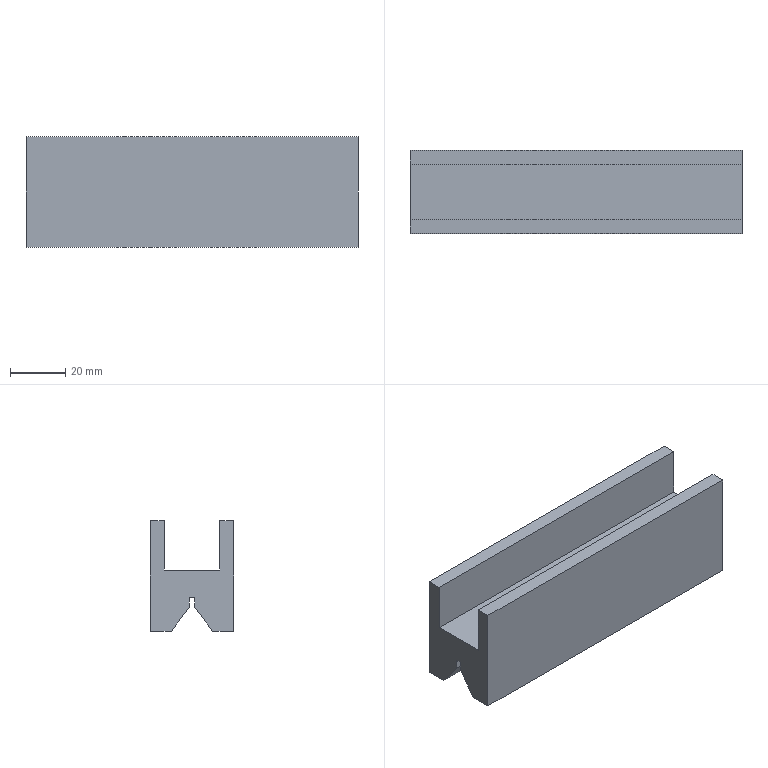CAM job | Mastercam | mm | 8 operations | part box 120 x 30 x 40
1. Contour (Ramp) | 2 - 12 平铣刀
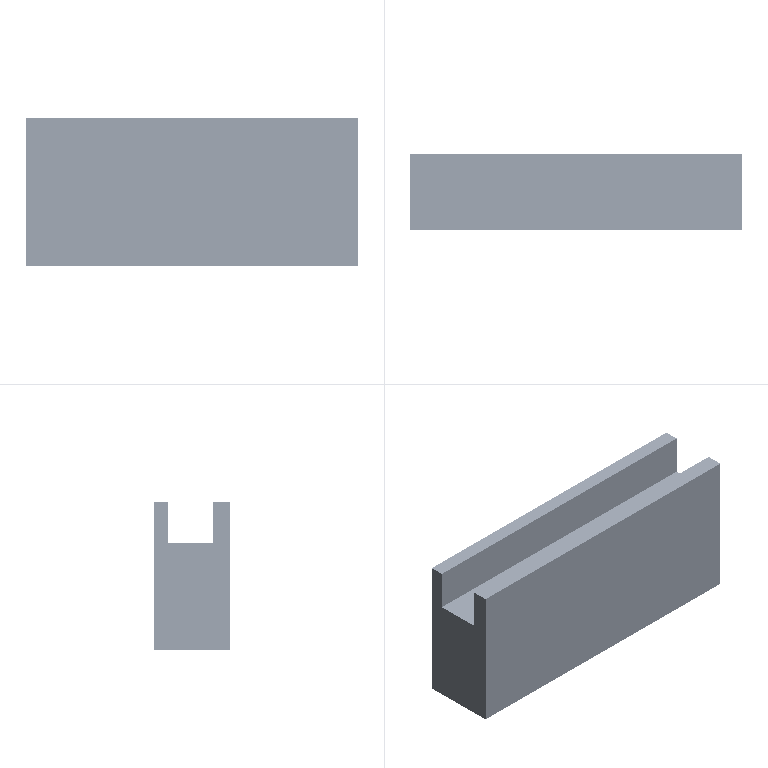2. Contour (2D) | 3 - 12 平铣刀
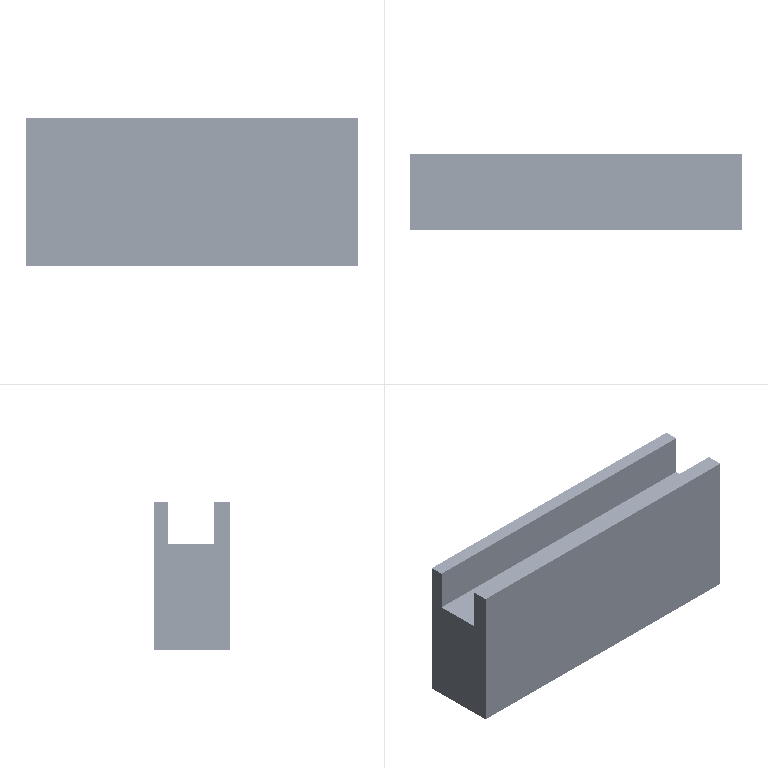3. Model Chamfer | 6 - 6 倒角刀
4. Surface Rough Pocket | 8 - 4 平铣刀
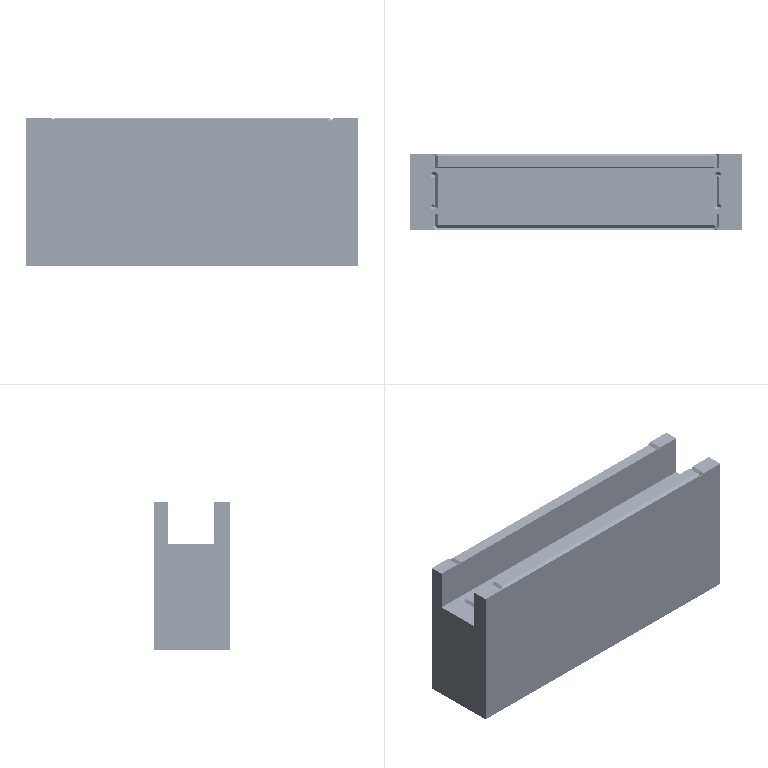5. 3D High Speed (Area roughing) | 17 - 2 平铣刀
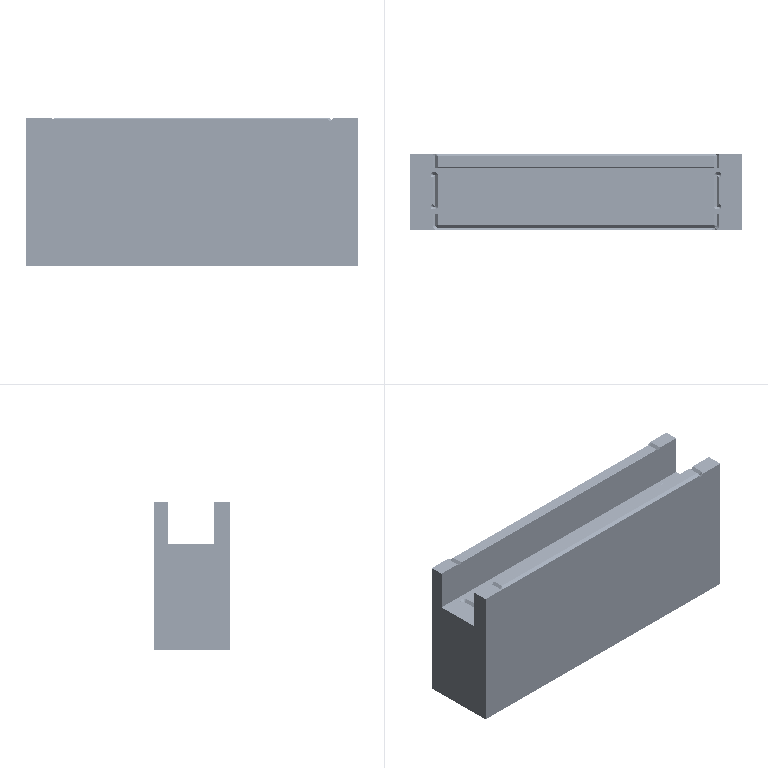6. Contour (Ramp) | 17 - 2 平铣刀
7. Contour (2D) | 18 - 2 平铣刀
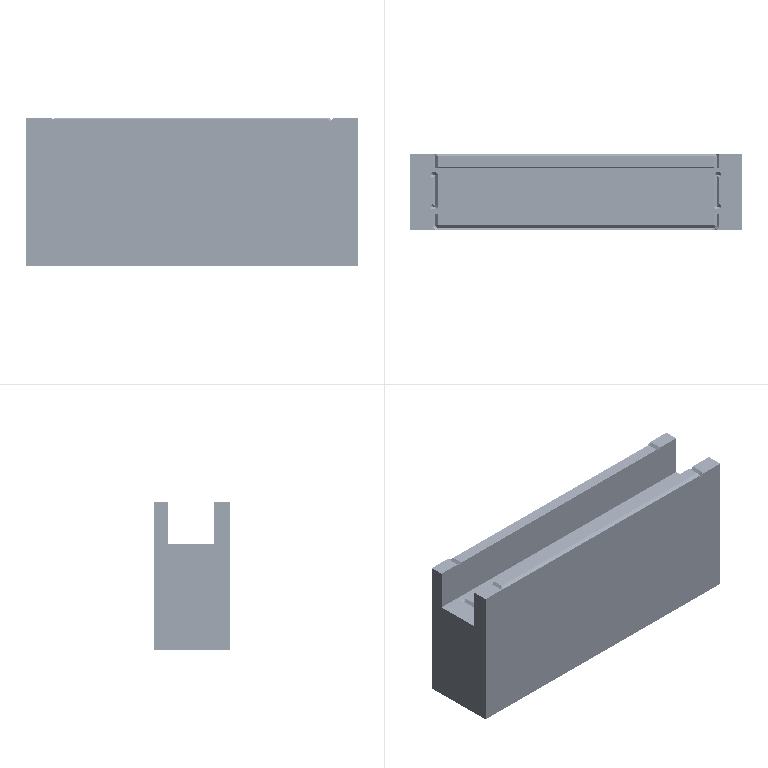8. Surface Finish Flowline | 21 - 2 圆鼻铣刀